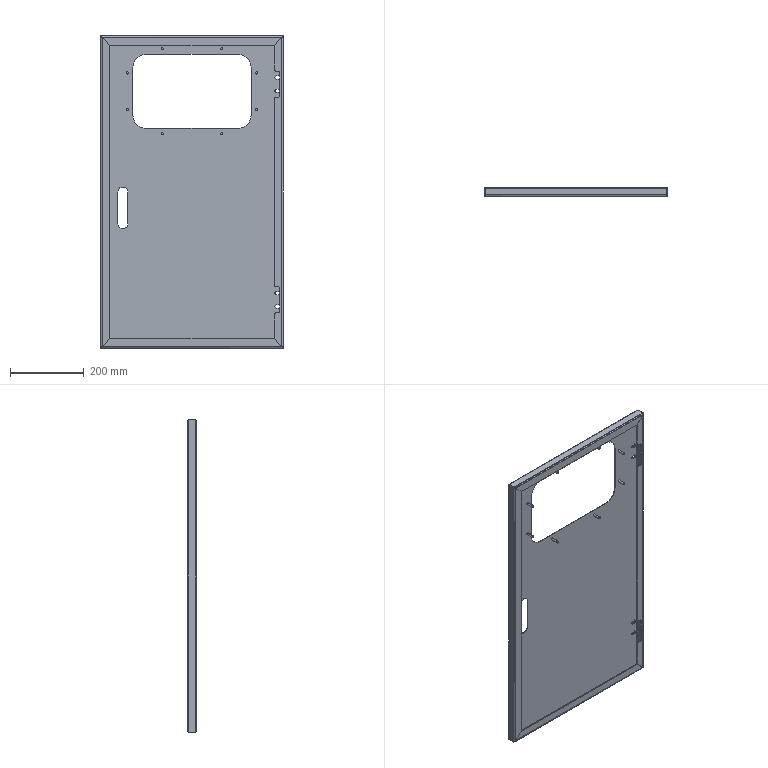Component | SolidWorks | ElectricalCabinetDoorAssembly-1_ElectricalCabinetDoor-1 | 1 solid | 142 faces | volume 931680 mm3 | plane 68 | cylinder 58 | spline 16 | commonest cylinder face diameters 6 x16 9 x12 4 x8 8 x8 10 x8 70 x4 26.5 x2 | material Plain Carbon Steel